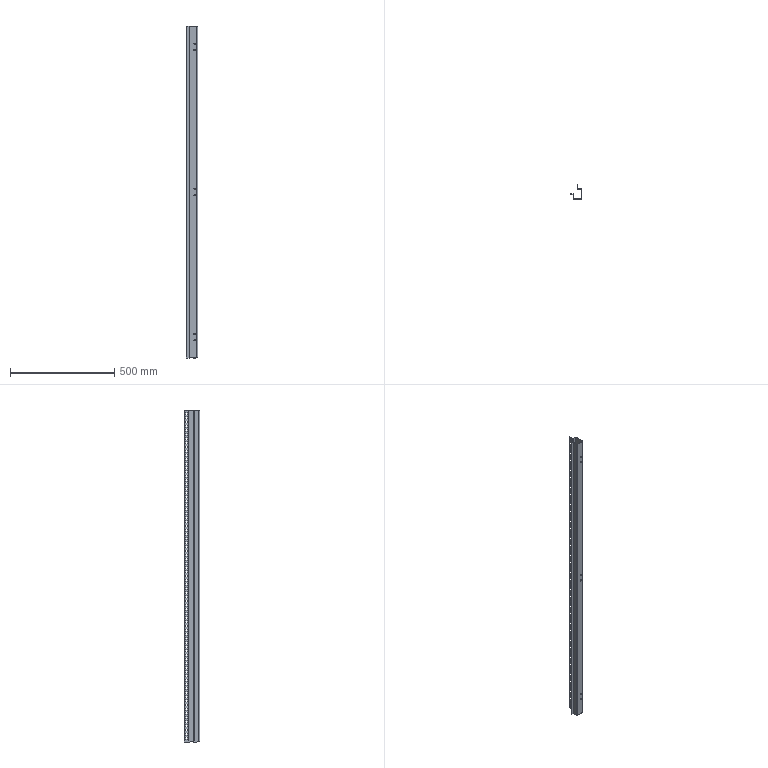Component | SolidWorks | LeftColumn-1 | 1 solid | 374 faces | volume 509091 mm3 | plane 352 | cylinder 22 | commonest cylinder face diameters 6 x17 2 x5